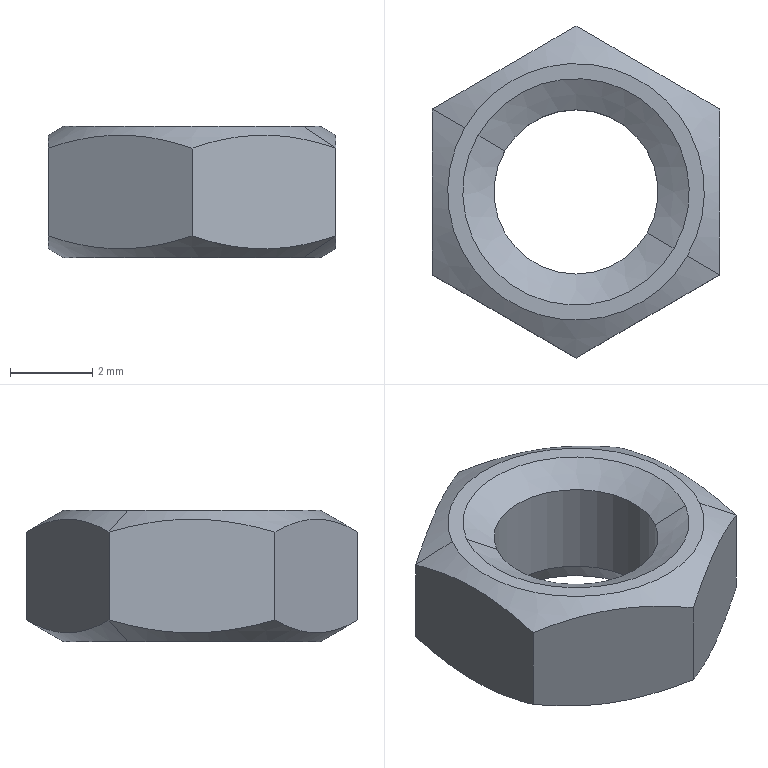Component | SolidWorks | M4-3 | 1 solid | 18 faces | box 7 x 8.08 x 3.2 mm | volume 88 mm3 | cone 8 | plane 8 | cylinder 2 | commonest cylinder face diameters 4 x2 | material Standard Part
STEP:
#1=CARTESIAN_POINT('',(-0.734,0.3859,-1.071));
#2=VERTEX_POINT('',#1);
#3=CARTESIAN_POINT('',(-0.9471,0.5089,-1.071));
#4=VERTEX_POINT('',#3);
#5=CARTESIAN_POINT('',(-0.8406,0.4474,-1.071));
#6=DIRECTION('',(-0.,-0.,1.));
#7=DIRECTION('',(0.866,-0.5,0.));
#8=AXIS2_PLACEMENT_3D('',#5,#6,#7);
#9=CIRCLE('',#8,0.123);
#10=EDGE_CURVE('',#2,#4,#9,.T.);
#11=ORIENTED_EDGE('',*,*,#10,.T.);
#12=CARTESIAN_POINT('',(-0.9784,0.527,-1.05));
#13=VERTEX_POINT('',#12);
#14=CARTESIAN_POINT('',(-0.9786,0.5271,-1.05));
#15=DIRECTION('',(-0.75,0.433,0.5));
#16=VECTOR('',#15,39.37);
#17=LINE('',#14,#16);
#18=EDGE_CURVE('',#4,#13,#17,.T.);
#19=ORIENTED_EDGE('',*,*,#18,.T.);
#20=CARTESIAN_POINT('',(-0.8406,0.6065,-1.05));
#21=VERTEX_POINT('',#20);
#22=CARTESIAN_POINT('',(-0.9784,0.527,-1.05));
#23=CARTESIAN_POINT('',(-0.9559,0.54,-1.058));
#24=CARTESIAN_POINT('',(-0.933,0.5531,-1.062));
#25=CARTESIAN_POINT('',(-0.8979,0.5734,-1.062));
#26=CARTESIAN_POINT('',(-0.8862,0.5802,-1.061));
#27=CARTESIAN_POINT('',(-0.8632,0.5935,-1.057));
#28=CARTESIAN_POINT('',(-0.8518,0.6,-1.054));
#29=CARTESIAN_POINT('',(-0.8406,0.6065,-1.05));
#30=B_SPLINE_CURVE_WITH_KNOTS('',3,(#22,#23,#24,#25,#26,#27,#28,#29),.UNSPECIFIED.,.F.,.F.,(4,2,2,4),(0.,0.002041,0.003061,0.004082),.UNSPECIFIED.);
#31=EDGE_CURVE('',#13,#21,#30,.T.);
#32=ORIENTED_EDGE('',*,*,#31,.T.);
#33=CARTESIAN_POINT('',(-0.7028,0.527,-1.05));
#34=VERTEX_POINT('',#33);
#35=CARTESIAN_POINT('',(-0.8406,0.6065,-1.05));
#36=CARTESIAN_POINT('',(-0.8181,0.5935,-1.058));
#37=CARTESIAN_POINT('',(-0.7952,0.5804,-1.062));
#38=CARTESIAN_POINT('',(-0.7601,0.5601,-1.062));
#39=CARTESIAN_POINT('',(-0.7484,0.5533,-1.061));
#40=CARTESIAN_POINT('',(-0.7254,0.54,-1.057));
#41=CARTESIAN_POINT('',(-0.714,0.5335,-1.054));
#42=CARTESIAN_POINT('',(-0.7028,0.527,-1.05));
#43=B_SPLINE_CURVE_WITH_KNOTS('',3,(#35,#36,#37,#38,#39,#40,#41,#42),.UNSPECIFIED.,.F.,.F.,(4,2,2,4),(0.,0.002041,0.003061,0.004082),.UNSPECIFIED.);
#44=EDGE_CURVE('',#21,#34,#43,.T.);
#45=ORIENTED_EDGE('',*,*,#44,.T.);
#46=CARTESIAN_POINT('',(-0.7028,0.3679,-1.05));
#47=VERTEX_POINT('',#46);
#48=CARTESIAN_POINT('',(-0.7028,0.527,-1.05));
#49=CARTESIAN_POINT('',(-0.7028,0.501,-1.058));
#50=CARTESIAN_POINT('',(-0.7028,0.4746,-1.062));
#51=CARTESIAN_POINT('',(-0.7028,0.434,-1.062));
#52=CARTESIAN_POINT('',(-0.7028,0.4205,-1.061));
#53=CARTESIAN_POINT('',(-0.7028,0.394,-1.057));
#54=CARTESIAN_POINT('',(-0.7028,0.3809,-1.054));
#55=CARTESIAN_POINT('',(-0.7028,0.3679,-1.05));
#56=B_SPLINE_CURVE_WITH_KNOTS('',3,(#48,#49,#50,#51,#52,#53,#54,#55),.UNSPECIFIED.,.F.,.F.,(4,2,2,4),(0.,0.002041,0.003061,0.004082),.UNSPECIFIED.);
#57=EDGE_CURVE('',#34,#47,#56,.T.);
#58=ORIENTED_EDGE('',*,*,#57,.T.);
#59=CARTESIAN_POINT('',(-0.7026,0.3677,-1.05));
#60=DIRECTION('',(0.75,-0.433,0.5));
#61=VECTOR('',#60,39.37);
#62=LINE('',#59,#61);
#63=EDGE_CURVE('',#2,#47,#62,.T.);
#64=ORIENTED_EDGE('',*,*,#63,.F.);
#65=EDGE_LOOP('',(#11,#19,#32,#45,#58,#64));
#66=FACE_OUTER_BOUND('',#65,.T.);
#67=CARTESIAN_POINT('',(-0.8406,0.4474,-1.05));
#68=DIRECTION('',(-0.,-0.,1.));
#69=DIRECTION('',(0.866,-0.5,0.));
#70=AXIS2_PLACEMENT_3D('',#67,#68,#69);
#71=CONICAL_SURFACE('',#70,0.1593,1.047);
#72=ADVANCED_FACE('',(#66),#71,.T.);
#73=CARTESIAN_POINT('',(-0.7724,0.408,-1.052));
#74=VERTEX_POINT('',#73);
#75=CARTESIAN_POINT('',(-0.9088,0.4868,-1.052));
#76=VERTEX_POINT('',#75);
#77=CARTESIAN_POINT('',(-0.8406,0.4474,-1.052));
#78=DIRECTION('',(0.,0.,-1.));
#79=DIRECTION('',(-0.866,0.5,0.));
#80=AXIS2_PLACEMENT_3D('',#77,#78,#79);
#81=CIRCLE('',#80,0.07874);
#82=EDGE_CURVE('',#74,#76,#81,.T.);
#83=ORIENTED_EDGE('',*,*,#82,.F.);
#84=CARTESIAN_POINT('',(-0.7629,0.4026,-1.071));
#85=VERTEX_POINT('',#84);
#86=CARTESIAN_POINT('',(-0.7667,0.4047,-1.063));
#87=DIRECTION('',(0.433,-0.25,-0.866));
#88=VECTOR('',#87,39.37);
#89=LINE('',#86,#88);
#90=EDGE_CURVE('',#74,#85,#89,.T.);
#91=ORIENTED_EDGE('',*,*,#90,.T.);
#92=CARTESIAN_POINT('',(-0.9182,0.4922,-1.071));
#93=VERTEX_POINT('',#92);
#94=CARTESIAN_POINT('',(-0.8406,0.4474,-1.071));
#95=DIRECTION('',(0.,0.,-1.));
#96=DIRECTION('',(0.866,-0.5,0.));
#97=AXIS2_PLACEMENT_3D('',#94,#95,#96);
#98=CIRCLE('',#97,0.08966);
#99=EDGE_CURVE('',#85,#93,#98,.T.);
#100=ORIENTED_EDGE('',*,*,#99,.T.);
#101=CARTESIAN_POINT('',(-0.9145,0.4901,-1.063));
#102=DIRECTION('',(-0.433,0.25,-0.866));
#103=VECTOR('',#102,39.37);
#104=LINE('',#101,#103);
#105=EDGE_CURVE('',#76,#93,#104,.T.);
#106=ORIENTED_EDGE('',*,*,#105,.F.);
#107=EDGE_LOOP('',(#83,#91,#100,#106));
#108=FACE_OUTER_BOUND('',#107,.T.);
#109=CARTESIAN_POINT('',(-0.8406,0.4474,-1.063));
#110=DIRECTION('',(0.,0.,-1.));
#111=DIRECTION('',(-0.866,0.5,0.));
#112=AXIS2_PLACEMENT_3D('',#109,#110,#111);
#113=CONICAL_SURFACE('',#112,0.08536,0.5236);
#114=ADVANCED_FACE('',(#108),#113,.F.);
#115=ORIENTED_EDGE('',*,*,#82,.T.);
#116=CARTESIAN_POINT('',(-0.9088,0.4868,-0.9621));
#117=VERTEX_POINT('',#116);
#118=CARTESIAN_POINT('',(-0.9088,0.4868,-1.071));
#119=DIRECTION('',(-0.,-0.,1.));
#120=VECTOR('',#119,39.37);
#121=LINE('',#118,#120);
#122=EDGE_CURVE('',#76,#117,#121,.T.);
#123=ORIENTED_EDGE('',*,*,#122,.T.);
#124=CARTESIAN_POINT('',(-0.7724,0.408,-0.9621));
#125=VERTEX_POINT('',#124);
#126=CARTESIAN_POINT('',(-0.8406,0.4474,-0.9621));
#127=DIRECTION('',(0.,0.,-1.));
#128=DIRECTION('',(0.866,-0.5,0.));
#129=AXIS2_PLACEMENT_3D('',#126,#127,#128);
#130=CIRCLE('',#129,0.07874);
#131=EDGE_CURVE('',#125,#117,#130,.T.);
#132=ORIENTED_EDGE('',*,*,#131,.F.);
#133=CARTESIAN_POINT('',(-0.7724,0.408,-1.071));
#134=DIRECTION('',(-0.,-0.,1.));
#135=VECTOR('',#134,39.37);
#136=LINE('',#133,#135);
#137=EDGE_CURVE('',#74,#125,#136,.T.);
#138=ORIENTED_EDGE('',*,*,#137,.F.);
#139=EDGE_LOOP('',(#115,#123,#132,#138));
#140=FACE_OUTER_BOUND('',#139,.T.);
#141=CARTESIAN_POINT('',(-0.8406,0.4474,-1.071));
#142=DIRECTION('',(-0.,-0.,1.));
#143=DIRECTION('',(0.866,-0.5,0.));
#144=AXIS2_PLACEMENT_3D('',#141,#142,#143);
#145=CYLINDRICAL_SURFACE('',#144,0.07874);
#146=ADVANCED_FACE('',(#140),#145,.F.);
#147=CARTESIAN_POINT('',(-0.9471,0.5089,-0.9449));
#148=VERTEX_POINT('',#147);
#149=CARTESIAN_POINT('',(-0.734,0.3859,-0.9449));
#150=VERTEX_POINT('',#149);
#151=CARTESIAN_POINT('',(-0.8406,0.4474,-0.9449));
#152=DIRECTION('',(0.,0.,-1.));
#153=DIRECTION('',(-0.866,0.5,0.));
#154=AXIS2_PLACEMENT_3D('',#151,#152,#153);
#155=CIRCLE('',#154,0.123);
#156=EDGE_CURVE('',#148,#150,#155,.T.);
#157=ORIENTED_EDGE('',*,*,#156,.T.);
#158=CARTESIAN_POINT('',(-0.7028,0.3679,-0.9657));
#159=VERTEX_POINT('',#158);
#160=CARTESIAN_POINT('',(-0.7026,0.3677,-0.9658));
#161=DIRECTION('',(0.75,-0.433,-0.5));
#162=VECTOR('',#161,39.37);
#163=LINE('',#160,#162);
#164=EDGE_CURVE('',#150,#159,#163,.T.);
#165=ORIENTED_EDGE('',*,*,#164,.T.);
#166=CARTESIAN_POINT('',(-0.7028,0.527,-0.9657));
#167=VERTEX_POINT('',#166);
#168=CARTESIAN_POINT('',(-0.7028,0.527,-0.9657));
#169=CARTESIAN_POINT('',(-0.7028,0.501,-0.9582));
#170=CARTESIAN_POINT('',(-0.7028,0.4746,-0.9534));
#171=CARTESIAN_POINT('',(-0.7028,0.434,-0.9534));
#172=CARTESIAN_POINT('',(-0.7028,0.4205,-0.9546));
#173=CARTESIAN_POINT('',(-0.7028,0.394,-0.9589));
#174=CARTESIAN_POINT('',(-0.7028,0.3809,-0.962));
#175=CARTESIAN_POINT('',(-0.7028,0.3679,-0.9657));
#176=B_SPLINE_CURVE_WITH_KNOTS('',3,(#168,#169,#170,#171,#172,#173,#174,#175),.UNSPECIFIED.,.F.,.F.,(4,2,2,4),(0.,0.002041,0.003061,0.004082),.UNSPECIFIED.);
#177=EDGE_CURVE('',#167,#159,#176,.T.);
#178=ORIENTED_EDGE('',*,*,#177,.F.);
#179=CARTESIAN_POINT('',(-0.8406,0.6065,-0.9657));
#180=VERTEX_POINT('',#179);
#181=CARTESIAN_POINT('',(-0.8406,0.6065,-0.9657));
#182=CARTESIAN_POINT('',(-0.8181,0.5935,-0.9582));
#183=CARTESIAN_POINT('',(-0.7952,0.5804,-0.9534));
#184=CARTESIAN_POINT('',(-0.7601,0.5601,-0.9534));
#185=CARTESIAN_POINT('',(-0.7484,0.5533,-0.9546));
#186=CARTESIAN_POINT('',(-0.7254,0.54,-0.9589));
#187=CARTESIAN_POINT('',(-0.714,0.5335,-0.962));
#188=CARTESIAN_POINT('',(-0.7028,0.527,-0.9657));
#189=B_SPLINE_CURVE_WITH_KNOTS('',3,(#181,#182,#183,#184,#185,#186,#187,#188),.UNSPECIFIED.,.F.,.F.,(4,2,2,4),(0.,0.002041,0.003061,0.004082),.UNSPECIFIED.);
#190=EDGE_CURVE('',#180,#167,#189,.T.);
#191=ORIENTED_EDGE('',*,*,#190,.F.);
#192=CARTESIAN_POINT('',(-0.9784,0.527,-0.9657));
#193=VERTEX_POINT('',#192);
#194=CARTESIAN_POINT('',(-0.9784,0.527,-0.9657));
#195=CARTESIAN_POINT('',(-0.9559,0.54,-0.9582));
#196=CARTESIAN_POINT('',(-0.933,0.5531,-0.9534));
#197=CARTESIAN_POINT('',(-0.8979,0.5734,-0.9534));
#198=CARTESIAN_POINT('',(-0.8862,0.5802,-0.9546));
#199=CARTESIAN_POINT('',(-0.8632,0.5935,-0.9589));
#200=CARTESIAN_POINT('',(-0.8518,0.6,-0.962));
#201=CARTESIAN_POINT('',(-0.8406,0.6065,-0.9657));
#202=B_SPLINE_CURVE_WITH_KNOTS('',3,(#194,#195,#196,#197,#198,#199,#200,#201),.UNSPECIFIED.,.F.,.F.,(4,2,2,4),(0.,0.002041,0.003061,0.004082),.UNSPECIFIED.);
#203=EDGE_CURVE('',#193,#180,#202,.T.);
#204=ORIENTED_EDGE('',*,*,#203,.F.);
#205=CARTESIAN_POINT('',(-0.9786,0.5271,-0.9658));
#206=DIRECTION('',(-0.75,0.433,-0.5));
#207=VECTOR('',#206,39.37);
#208=LINE('',#205,#207);
#209=EDGE_CURVE('',#148,#193,#208,.T.);
#210=ORIENTED_EDGE('',*,*,#209,.F.);
#211=EDGE_LOOP('',(#157,#165,#178,#191,#204,#210));
#212=FACE_OUTER_BOUND('',#211,.T.);
#213=CARTESIAN_POINT('',(-0.8406,0.4474,-0.9658));
#214=DIRECTION('',(0.,0.,-1.));
#215=DIRECTION('',(-0.866,0.5,0.));
#216=AXIS2_PLACEMENT_3D('',#213,#214,#215);
#217=CONICAL_SURFACE('',#216,0.1593,1.047);
#218=ADVANCED_FACE('',(#212),#217,.T.);
#219=ORIENTED_EDGE('',*,*,#131,.T.);
#220=CARTESIAN_POINT('',(-0.9346,0.5017,-0.9449));
#221=VERTEX_POINT('',#220);
#222=CARTESIAN_POINT('',(-0.9152,0.4905,-0.9578));
#223=DIRECTION('',(-0.75,0.433,0.5));
#224=VECTOR('',#223,39.37);
#225=LINE('',#222,#224);
#226=EDGE_CURVE('',#117,#221,#225,.T.);
#227=ORIENTED_EDGE('',*,*,#226,.T.);
#228=CARTESIAN_POINT('',(-0.7465,0.3931,-0.9449));
#229=VERTEX_POINT('',#228);
#230=CARTESIAN_POINT('',(-0.8406,0.4474,-0.9449));
#231=DIRECTION('',(0.,0.,-1.));
#232=DIRECTION('',(0.866,-0.5,0.));
#233=AXIS2_PLACEMENT_3D('',#230,#231,#232);
#234=CIRCLE('',#233,0.1086);
#235=EDGE_CURVE('',#229,#221,#234,.T.);
#236=ORIENTED_EDGE('',*,*,#235,.F.);
#237=CARTESIAN_POINT('',(-0.7659,0.4043,-0.9578));
#238=DIRECTION('',(0.75,-0.433,0.5));
#239=VECTOR('',#238,39.37);
#240=LINE('',#237,#239);
#241=EDGE_CURVE('',#125,#229,#240,.T.);
#242=ORIENTED_EDGE('',*,*,#241,.F.);
#243=EDGE_LOOP('',(#219,#227,#236,#242));
#244=FACE_OUTER_BOUND('',#243,.T.);
#245=CARTESIAN_POINT('',(-0.8406,0.4474,-0.9578));
#246=DIRECTION('',(-0.,-0.,1.));
#247=DIRECTION('',(0.866,-0.5,0.));
#248=AXIS2_PLACEMENT_3D('',#245,#246,#247);
#249=CONICAL_SURFACE('',#248,0.0862,1.047);
#250=ADVANCED_FACE('',(#244),#249,.F.);
#251=ORIENTED_EDGE('',*,*,#10,.F.);
#252=CARTESIAN_POINT('',(-0.8406,0.4474,-1.071));
#253=DIRECTION('',(-0.,-0.,1.));
#254=DIRECTION('',(0.866,-0.5,0.));
#255=AXIS2_PLACEMENT_3D('',#252,#253,#254);
#256=CIRCLE('',#255,0.123);
#257=EDGE_CURVE('',#4,#2,#256,.T.);
#258=ORIENTED_EDGE('',*,*,#257,.F.);
#259=EDGE_LOOP('',(#251,#258));
#260=FACE_OUTER_BOUND('',#259,.T.);
#261=CARTESIAN_POINT('',(-0.8406,0.4474,-1.071));
#262=DIRECTION('',(0.,0.,-1.));
#263=DIRECTION('',(0.866,-0.5,0.));
#264=AXIS2_PLACEMENT_3D('',#261,#262,#263);
#265=CIRCLE('',#264,0.08966);
#266=EDGE_CURVE('',#93,#85,#265,.T.);
#267=ORIENTED_EDGE('',*,*,#266,.F.);
#268=ORIENTED_EDGE('',*,*,#99,.F.);
#269=EDGE_LOOP('',(#267,#268));
#270=FACE_BOUND('',#269,.T.);
#271=CARTESIAN_POINT('',(-0.7028,0.3679,-1.071));
#272=DIRECTION('',(-0.,-0.,1.));
#273=DIRECTION('',(0.866,-0.5,0.));
#274=AXIS2_PLACEMENT_3D('',#271,#272,#273);
#275=PLANE('',#274);
#276=ADVANCED_FACE('',(#260,#270),#275,.F.);
#277=ORIENTED_EDGE('',*,*,#18,.F.);
#278=ORIENTED_EDGE('',*,*,#257,.T.);
#279=ORIENTED_EDGE('',*,*,#63,.T.);
#280=CARTESIAN_POINT('',(-0.8406,0.2883,-1.05));
#281=VERTEX_POINT('',#280);
#282=CARTESIAN_POINT('',(-0.7028,0.3679,-1.05));
#283=CARTESIAN_POINT('',(-0.7253,0.3549,-1.058));
#284=CARTESIAN_POINT('',(-0.7481,0.3417,-1.062));
#285=CARTESIAN_POINT('',(-0.7833,0.3214,-1.062));
#286=CARTESIAN_POINT('',(-0.795,0.3146,-1.061));
#287=CARTESIAN_POINT('',(-0.818,0.3014,-1.057));
#288=CARTESIAN_POINT('',(-0.8293,0.2948,-1.054));
#289=CARTESIAN_POINT('',(-0.8406,0.2883,-1.05));
#290=B_SPLINE_CURVE_WITH_KNOTS('',3,(#282,#283,#284,#285,#286,#287,#288,#289),.UNSPECIFIED.,.F.,.F.,(4,2,2,4),(0.,0.002041,0.003061,0.004082),.UNSPECIFIED.);
#291=EDGE_CURVE('',#47,#281,#290,.T.);
#292=ORIENTED_EDGE('',*,*,#291,.T.);
#293=CARTESIAN_POINT('',(-0.9784,0.3679,-1.05));
#294=VERTEX_POINT('',#293);
#295=CARTESIAN_POINT('',(-0.8406,0.2883,-1.05));
#296=CARTESIAN_POINT('',(-0.8631,0.3013,-1.058));
#297=CARTESIAN_POINT('',(-0.8859,0.3145,-1.062));
#298=CARTESIAN_POINT('',(-0.9211,0.3348,-1.062));
#299=CARTESIAN_POINT('',(-0.9328,0.3415,-1.061));
#300=CARTESIAN_POINT('',(-0.9558,0.3548,-1.057));
#301=CARTESIAN_POINT('',(-0.9671,0.3614,-1.054));
#302=CARTESIAN_POINT('',(-0.9784,0.3679,-1.05));
#303=B_SPLINE_CURVE_WITH_KNOTS('',3,(#295,#296,#297,#298,#299,#300,#301,#302),.UNSPECIFIED.,.F.,.F.,(4,2,2,4),(0.,0.002041,0.003061,0.004082),.UNSPECIFIED.);
#304=EDGE_CURVE('',#281,#294,#303,.T.);
#305=ORIENTED_EDGE('',*,*,#304,.T.);
#306=CARTESIAN_POINT('',(-0.9784,0.3679,-1.05));
#307=CARTESIAN_POINT('',(-0.9784,0.3938,-1.058));
#308=CARTESIAN_POINT('',(-0.9784,0.4202,-1.062));
#309=CARTESIAN_POINT('',(-0.9784,0.4608,-1.062));
#310=CARTESIAN_POINT('',(-0.9784,0.4743,-1.061));
#311=CARTESIAN_POINT('',(-0.9784,0.5008,-1.057));
#312=CARTESIAN_POINT('',(-0.9784,0.514,-1.054));
#313=CARTESIAN_POINT('',(-0.9784,0.527,-1.05));
#314=B_SPLINE_CURVE_WITH_KNOTS('',3,(#306,#307,#308,#309,#310,#311,#312,#313),.UNSPECIFIED.,.F.,.F.,(4,2,2,4),(0.,0.002041,0.003061,0.004082),.UNSPECIFIED.);
#315=EDGE_CURVE('',#294,#13,#314,.T.);
#316=ORIENTED_EDGE('',*,*,#315,.T.);
#317=EDGE_LOOP('',(#277,#278,#279,#292,#305,#316));
#318=FACE_OUTER_BOUND('',#317,.T.);
#319=CARTESIAN_POINT('',(-0.8406,0.4474,-1.05));
#320=DIRECTION('',(-0.,-0.,1.));
#321=DIRECTION('',(0.866,-0.5,0.));
#322=AXIS2_PLACEMENT_3D('',#319,#320,#321);
#323=CONICAL_SURFACE('',#322,0.1593,1.047);
#324=ADVANCED_FACE('',(#318),#323,.T.);
#325=ORIENTED_EDGE('',*,*,#90,.F.);
#326=CARTESIAN_POINT('',(-0.8406,0.4474,-1.052));
#327=DIRECTION('',(0.,0.,-1.));
#328=DIRECTION('',(-0.866,0.5,0.));
#329=AXIS2_PLACEMENT_3D('',#326,#327,#328);
#330=CIRCLE('',#329,0.07874);
#331=EDGE_CURVE('',#76,#74,#330,.T.);
#332=ORIENTED_EDGE('',*,*,#331,.F.);
#333=ORIENTED_EDGE('',*,*,#105,.T.);
#334=ORIENTED_EDGE('',*,*,#266,.T.);
#335=EDGE_LOOP('',(#325,#332,#333,#334));
#336=FACE_OUTER_BOUND('',#335,.T.);
#337=CARTESIAN_POINT('',(-0.8406,0.4474,-1.063));
#338=DIRECTION('',(0.,0.,-1.));
#339=DIRECTION('',(-0.866,0.5,0.));
#340=AXIS2_PLACEMENT_3D('',#337,#338,#339);
#341=CONICAL_SURFACE('',#340,0.08536,0.5236);
#342=ADVANCED_FACE('',(#336),#341,.F.);
#343=ORIENTED_EDGE('',*,*,#315,.F.);
#344=CARTESIAN_POINT('',(-0.9784,0.3679,-0.9657));
#345=VERTEX_POINT('',#344);
#346=CARTESIAN_POINT('',(-0.9784,0.3679,-1.071));
#347=DIRECTION('',(-0.,-0.,1.));
#348=VECTOR('',#347,39.37);
#349=LINE('',#346,#348);
#350=EDGE_CURVE('',#294,#345,#349,.T.);
#351=ORIENTED_EDGE('',*,*,#350,.T.);
#352=CARTESIAN_POINT('',(-0.9784,0.3679,-0.9657));
#353=CARTESIAN_POINT('',(-0.9784,0.3938,-0.9582));
#354=CARTESIAN_POINT('',(-0.9784,0.4202,-0.9534));
#355=CARTESIAN_POINT('',(-0.9784,0.4608,-0.9534));
#356=CARTESIAN_POINT('',(-0.9784,0.4743,-0.9546));
#357=CARTESIAN_POINT('',(-0.9784,0.5008,-0.9589));
#358=CARTESIAN_POINT('',(-0.9784,0.514,-0.962));
#359=CARTESIAN_POINT('',(-0.9784,0.527,-0.9657));
#360=B_SPLINE_CURVE_WITH_KNOTS('',3,(#352,#353,#354,#355,#356,#357,#358,#359),.UNSPECIFIED.,.F.,.F.,(4,2,2,4),(0.,0.002041,0.003061,0.004082),.UNSPECIFIED.);
#361=EDGE_CURVE('',#345,#193,#360,.T.);
#362=ORIENTED_EDGE('',*,*,#361,.T.);
#363=CARTESIAN_POINT('',(-0.9784,0.527,-1.071));
#364=DIRECTION('',(0.,0.,-1.));
#365=VECTOR('',#364,39.37);
#366=LINE('',#363,#365);
#367=EDGE_CURVE('',#193,#13,#366,.T.);
#368=ORIENTED_EDGE('',*,*,#367,.T.);
#369=EDGE_LOOP('',(#343,#351,#362,#368));
#370=FACE_OUTER_BOUND('',#369,.T.);
#371=CARTESIAN_POINT('',(-0.9784,0.527,-1.071));
#372=DIRECTION('',(-1.,0.,-0.));
#373=DIRECTION('',(-0.,-1.,-0.));
#374=AXIS2_PLACEMENT_3D('',#371,#372,#373);
#375=PLANE('',#374);
#376=ADVANCED_FACE('',(#370),#375,.T.);
#377=ORIENTED_EDGE('',*,*,#304,.F.);
#378=CARTESIAN_POINT('',(-0.8406,0.2883,-0.9657));
#379=VERTEX_POINT('',#378);
#380=CARTESIAN_POINT('',(-0.8406,0.2883,-1.071));
#381=DIRECTION('',(-0.,-0.,1.));
#382=VECTOR('',#381,39.37);
#383=LINE('',#380,#382);
#384=EDGE_CURVE('',#281,#379,#383,.T.);
#385=ORIENTED_EDGE('',*,*,#384,.T.);
#386=CARTESIAN_POINT('',(-0.8406,0.2883,-0.9657));
#387=CARTESIAN_POINT('',(-0.8631,0.3013,-0.9582));
#388=CARTESIAN_POINT('',(-0.8859,0.3145,-0.9534));
#389=CARTESIAN_POINT('',(-0.9211,0.3348,-0.9534));
#390=CARTESIAN_POINT('',(-0.9328,0.3415,-0.9546));
#391=CARTESIAN_POINT('',(-0.9558,0.3548,-0.9589));
#392=CARTESIAN_POINT('',(-0.9671,0.3614,-0.962));
#393=CARTESIAN_POINT('',(-0.9784,0.3679,-0.9657));
#394=B_SPLINE_CURVE_WITH_KNOTS('',3,(#386,#387,#388,#389,#390,#391,#392,#393),.UNSPECIFIED.,.F.,.F.,(4,2,2,4),(0.,0.002041,0.003061,0.004082),.UNSPECIFIED.);
#395=EDGE_CURVE('',#379,#345,#394,.T.);
#396=ORIENTED_EDGE('',*,*,#395,.T.);
#397=ORIENTED_EDGE('',*,*,#350,.F.);
#398=EDGE_LOOP('',(#377,#385,#396,#397));
#399=FACE_OUTER_BOUND('',#398,.T.);
#400=CARTESIAN_POINT('',(-0.9784,0.3679,-1.071));
#401=DIRECTION('',(-0.5,-0.866,-0.));
#402=DIRECTION('',(0.866,-0.5,0.));
#403=AXIS2_PLACEMENT_3D('',#400,#401,#402);
#404=PLANE('',#403);
#405=ADVANCED_FACE('',(#399),#404,.T.);
#406=ORIENTED_EDGE('',*,*,#291,.F.);
#407=CARTESIAN_POINT('',(-0.7028,0.3679,-1.071));
#408=DIRECTION('',(-0.,-0.,1.));
#409=VECTOR('',#408,39.37);
#410=LINE('',#407,#409);
#411=EDGE_CURVE('',#47,#159,#410,.T.);
#412=ORIENTED_EDGE('',*,*,#411,.T.);
#413=CARTESIAN_POINT('',(-0.7028,0.3679,-0.9657));
#414=CARTESIAN_POINT('',(-0.7253,0.3549,-0.9582));
#415=CARTESIAN_POINT('',(-0.7481,0.3417,-0.9534));
#416=CARTESIAN_POINT('',(-0.7833,0.3214,-0.9534));
#417=CARTESIAN_POINT('',(-0.795,0.3146,-0.9546));
#418=CARTESIAN_POINT('',(-0.818,0.3014,-0.9589));
#419=CARTESIAN_POINT('',(-0.8293,0.2948,-0.962));
#420=CARTESIAN_POINT('',(-0.8406,0.2883,-0.9657));
#421=B_SPLINE_CURVE_WITH_KNOTS('',3,(#413,#414,#415,#416,#417,#418,#419,#420),.UNSPECIFIED.,.F.,.F.,(4,2,2,4),(0.,0.002041,0.003061,0.004082),.UNSPECIFIED.);
#422=EDGE_CURVE('',#159,#379,#421,.T.);
#423=ORIENTED_EDGE('',*,*,#422,.T.);
#424=ORIENTED_EDGE('',*,*,#384,.F.);
#425=EDGE_LOOP('',(#406,#412,#423,#424));
#426=FACE_OUTER_BOUND('',#425,.T.);
#427=CARTESIAN_POINT('',(-0.8406,0.2883,-1.071));
#428=DIRECTION('',(0.5,-0.866,0.));
#429=DIRECTION('',(0.866,0.5,0.));
#430=AXIS2_PLACEMENT_3D('',#427,#428,#429);
#431=PLANE('',#430);
#432=ADVANCED_FACE('',(#426),#431,.T.);
#433=ORIENTED_EDGE('',*,*,#57,.F.);
#434=CARTESIAN_POINT('',(-0.7028,0.527,-1.071));
#435=DIRECTION('',(-0.,-0.,1.));
#436=VECTOR('',#435,39.37);
#437=LINE('',#434,#436);
#438=EDGE_CURVE('',#34,#167,#437,.T.);
#439=ORIENTED_EDGE('',*,*,#438,.T.);
#440=ORIENTED_EDGE('',*,*,#177,.T.);
#441=ORIENTED_EDGE('',*,*,#411,.F.);
#442=EDGE_LOOP('',(#433,#439,#440,#441));
#443=FACE_OUTER_BOUND('',#442,.T.);
#444=CARTESIAN_POINT('',(-0.7028,0.3679,-1.071));
#445=DIRECTION('',(1.,-0.,0.));
#446=DIRECTION('',(0.,1.,0.));
#447=AXIS2_PLACEMENT_3D('',#444,#445,#446);
#448=PLANE('',#447);
#449=ADVANCED_FACE('',(#443),#448,.T.);
#450=ORIENTED_EDGE('',*,*,#44,.F.);
#451=CARTESIAN_POINT('',(-0.8406,0.6065,-1.071));
#452=DIRECTION('',(-0.,-0.,1.));
#453=VECTOR('',#452,39.37);
#454=LINE('',#451,#453);
#455=EDGE_CURVE('',#21,#180,#454,.T.);
#456=ORIENTED_EDGE('',*,*,#455,.T.);
#457=ORIENTED_EDGE('',*,*,#190,.T.);
#458=ORIENTED_EDGE('',*,*,#438,.F.);
#459=EDGE_LOOP('',(#450,#456,#457,#458));
#460=FACE_OUTER_BOUND('',#459,.T.);
#461=CARTESIAN_POINT('',(-0.7028,0.527,-1.071));
#462=DIRECTION('',(0.5,0.866,0.));
#463=DIRECTION('',(-0.,-0.,1.));
#464=AXIS2_PLACEMENT_3D('',#461,#462,#463);
#465=PLANE('',#464);
#466=ADVANCED_FACE('',(#460),#465,.T.);
#467=ORIENTED_EDGE('',*,*,#31,.F.);
#468=ORIENTED_EDGE('',*,*,#367,.F.);
#469=ORIENTED_EDGE('',*,*,#203,.T.);
#470=ORIENTED_EDGE('',*,*,#455,.F.);
#471=EDGE_LOOP('',(#467,#468,#469,#470));
#472=FACE_OUTER_BOUND('',#471,.T.);
#473=CARTESIAN_POINT('',(-0.8406,0.6065,-1.071));
#474=DIRECTION('',(-0.5,0.866,-0.));
#475=DIRECTION('',(-0.866,-0.5,-0.));
#476=AXIS2_PLACEMENT_3D('',#473,#474,#475);
#477=PLANE('',#476);
#478=ADVANCED_FACE('',(#472),#477,.T.);
#479=ORIENTED_EDGE('',*,*,#122,.F.);
#480=ORIENTED_EDGE('',*,*,#331,.T.);
#481=ORIENTED_EDGE('',*,*,#137,.T.);
#482=CARTESIAN_POINT('',(-0.8406,0.4474,-0.9621));
#483=DIRECTION('',(0.,0.,-1.));
#484=DIRECTION('',(0.866,-0.5,0.));
#485=AXIS2_PLACEMENT_3D('',#482,#483,#484);
#486=CIRCLE('',#485,0.07874);
#487=EDGE_CURVE('',#117,#125,#486,.T.);
#488=ORIENTED_EDGE('',*,*,#487,.F.);
#489=EDGE_LOOP('',(#479,#480,#481,#488));
#490=FACE_OUTER_BOUND('',#489,.T.);
#491=CARTESIAN_POINT('',(-0.8406,0.4474,-1.071));
#492=DIRECTION('',(-0.,-0.,1.));
#493=DIRECTION('',(0.866,-0.5,0.));
#494=AXIS2_PLACEMENT_3D('',#491,#492,#493);
#495=CYLINDRICAL_SURFACE('',#494,0.07874);
#496=ADVANCED_FACE('',(#490),#495,.F.);
#497=ORIENTED_EDGE('',*,*,#164,.F.);
#498=CARTESIAN_POINT('',(-0.8406,0.4474,-0.9449));
#499=DIRECTION('',(0.,0.,-1.));
#500=DIRECTION('',(-0.866,0.5,0.));
#501=AXIS2_PLACEMENT_3D('',#498,#499,#500);
#502=CIRCLE('',#501,0.123);
#503=EDGE_CURVE('',#150,#148,#502,.T.);
#504=ORIENTED_EDGE('',*,*,#503,.T.);
#505=ORIENTED_EDGE('',*,*,#209,.T.);
#506=ORIENTED_EDGE('',*,*,#361,.F.);
#507=ORIENTED_EDGE('',*,*,#395,.F.);
#508=ORIENTED_EDGE('',*,*,#422,.F.);
#509=EDGE_LOOP('',(#497,#504,#505,#506,#507,#508));
#510=FACE_OUTER_BOUND('',#509,.T.);
#511=CARTESIAN_POINT('',(-0.8406,0.4474,-0.9658));
#512=DIRECTION('',(0.,0.,-1.));
#513=DIRECTION('',(-0.866,0.5,0.));
#514=AXIS2_PLACEMENT_3D('',#511,#512,#513);
#515=CONICAL_SURFACE('',#514,0.1593,1.047);
#516=ADVANCED_FACE('',(#510),#515,.T.);
#517=ORIENTED_EDGE('',*,*,#226,.F.);
#518=ORIENTED_EDGE('',*,*,#487,.T.);
#519=ORIENTED_EDGE('',*,*,#241,.T.);
#520=CARTESIAN_POINT('',(-0.8406,0.4474,-0.9449));
#521=DIRECTION('',(0.,0.,-1.));
#522=DIRECTION('',(0.866,-0.5,0.));
#523=AXIS2_PLACEMENT_3D('',#520,#521,#522);
#524=CIRCLE('',#523,0.1086);
#525=EDGE_CURVE('',#221,#229,#524,.T.);
#526=ORIENTED_EDGE('',*,*,#525,.F.);
#527=EDGE_LOOP('',(#517,#518,#519,#526));
#528=FACE_OUTER_BOUND('',#527,.T.);
#529=CARTESIAN_POINT('',(-0.8406,0.4474,-0.9578));
#530=DIRECTION('',(-0.,-0.,1.));
#531=DIRECTION('',(0.866,-0.5,0.));
#532=AXIS2_PLACEMENT_3D('',#529,#530,#531);
#533=CONICAL_SURFACE('',#532,0.0862,1.047);
#534=ADVANCED_FACE('',(#528),#533,.F.);
#535=ORIENTED_EDGE('',*,*,#156,.F.);
#536=ORIENTED_EDGE('',*,*,#503,.F.);
#537=EDGE_LOOP('',(#535,#536));
#538=FACE_OUTER_BOUND('',#537,.T.);
#539=ORIENTED_EDGE('',*,*,#235,.T.);
#540=ORIENTED_EDGE('',*,*,#525,.T.);
#541=EDGE_LOOP('',(#539,#540));
#542=FACE_BOUND('',#541,.T.);
#543=CARTESIAN_POINT('',(-0.7028,0.3679,-0.9449));
#544=DIRECTION('',(-0.,-0.,1.));
#545=DIRECTION('',(0.866,-0.5,0.));
#546=AXIS2_PLACEMENT_3D('',#543,#544,#545);
#547=PLANE('',#546);
#548=ADVANCED_FACE('',(#538,#542),#547,.T.);
#549=CLOSED_SHELL('',(#72,#114,#146,#218,#250,#276,#324,#342,#376,#405,#432,#449,#466,#478,#496,#516,#534,#548));
#550=MANIFOLD_SOLID_BREP('',#549);
#551=CARTESIAN_POINT('',(0.,0.,0.));
#552=DIRECTION('',(0.,0.,1.));
#553=DIRECTION('',(1.,0.,0.));
#554=AXIS2_PLACEMENT_3D('',#551,#552,#553);
#555=(LENGTH_UNIT()NAMED_UNIT(*)SI_UNIT($,.METRE.));
#556=LENGTH_MEASURE_WITH_UNIT(LENGTH_MEASURE(0.0254),#555);
#557=DIMENSIONAL_EXPONENTS(1.,0.,0.,0.,0.,0.,0.);
#558=(CONVERSION_BASED_UNIT('',#556)LENGTH_UNIT()NAMED_UNIT(#557));
#559=UNCERTAINTY_MEASURE_WITH_UNIT(LENGTH_MEASURE(0.00001),#558,'','');
#560=(NAMED_UNIT(*)PLANE_ANGLE_UNIT()SI_UNIT($,.RADIAN.));
#561=(NAMED_UNIT(*)SI_UNIT($,.STERADIAN.)SOLID_ANGLE_UNIT());
#562=(GEOMETRIC_REPRESENTATION_CONTEXT(3)GLOBAL_UNCERTAINTY_ASSIGNED_CONTEXT((#559))GLOBAL_UNIT_ASSIGNED_CONTEXT((#558,#560,#561))REPRESENTATION_CONTEXT('',''));
#563=ADVANCED_BREP_SHAPE_REPRESENTATION('',(#550,#554),#562);
#564=COLOUR_RGB('',0.7922,0.8196,0.9333);
#565=FILL_AREA_STYLE_COLOUR('',#564);
#566=FILL_AREA_STYLE('',(#565));
#567=SURFACE_STYLE_FILL_AREA(#566);
#568=SURFACE_SIDE_STYLE('',(#567));
#569=SURFACE_STYLE_USAGE(.BOTH.,#568);
#570=PRESENTATION_STYLE_ASSIGNMENT((#569));
#571=STYLED_ITEM('',(#570),#550);
#572=(LENGTH_UNIT()NAMED_UNIT(*)SI_UNIT($,.METRE.));
#573=LENGTH_MEASURE_WITH_UNIT(LENGTH_MEASURE(0.0254),#572);
#574=DIMENSIONAL_EXPONENTS(1.,0.,0.,0.,0.,0.,0.);
#575=(CONVERSION_BASED_UNIT('',#573)LENGTH_UNIT()NAMED_UNIT(#574));
#576=UNCERTAINTY_MEASURE_WITH_UNIT(LENGTH_MEASURE(0.00001),#575,'','');
#577=(NAMED_UNIT(*)PLANE_ANGLE_UNIT()SI_UNIT($,.RADIAN.));
#578=(NAMED_UNIT(*)SI_UNIT($,.STERADIAN.)SOLID_ANGLE_UNIT());
#579=(GEOMETRIC_REPRESENTATION_CONTEXT(3)GLOBAL_UNCERTAINTY_ASSIGNED_CONTEXT((#576))GLOBAL_UNIT_ASSIGNED_CONTEXT((#575,#577,#578))REPRESENTATION_CONTEXT('',''));
#580=MECHANICAL_DESIGN_GEOMETRIC_PRESENTATION_REPRESENTATION('',(#571),#579);
#581=PRESENTATION_LAYER_ASSIGNMENT('','',(#571));